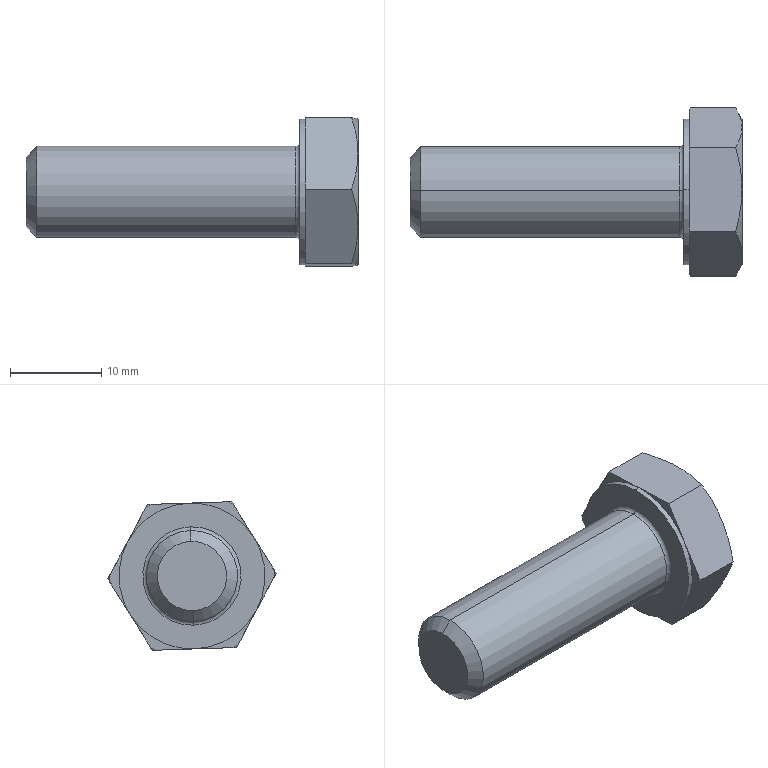Component | SolidWorks | GB_T5781-2000HexHeadBoltFullThreadC-gradeM10_30-1 | 1 solid | 35 faces | volume 3739 mm3 | plane 15 | cone 14 | cylinder 4 | torus 2 | commonest cylinder face diameters 10 x2 16 x2